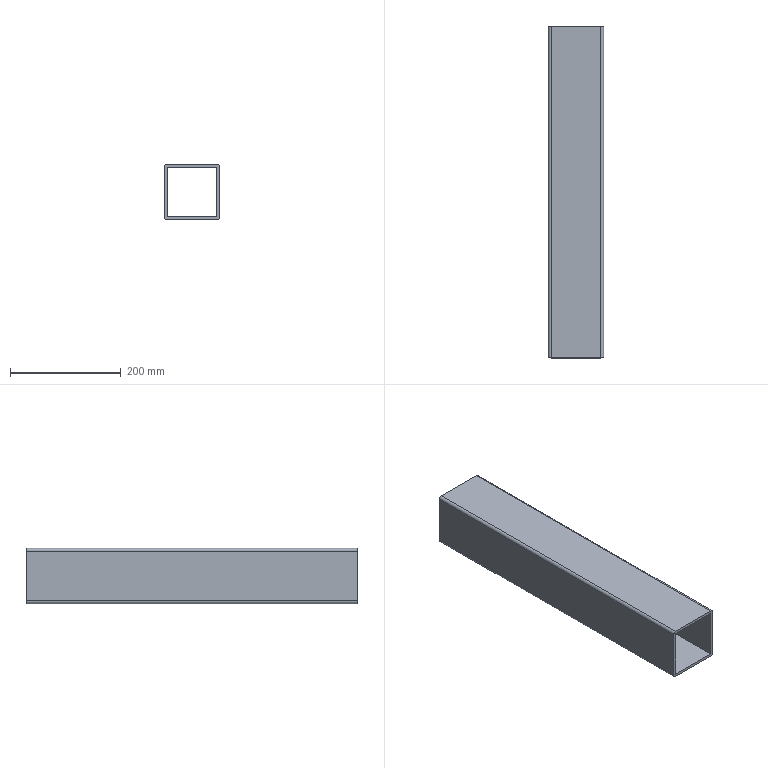Component | NX | TUBO_INFERIOR | 1 solid | 14 faces | box 100 x 600 x 100 mm | volume 1127124 mm3 | plane 10 | cylinder 4 | commonest cylinder face diameters 10 x4
STEP:
#1=CARTESIAN_POINT('',(0.,0.,0.));
#2=DIRECTION('',(0.,0.,1.));
#3=DIRECTION('',(1.,0.,0.));
#4=AXIS2_PLACEMENT_3D('',#1,#2,#3);
#5=CARTESIAN_POINT('',(0.,-34.8,155.));
#6=VERTEX_POINT('',#5);
#7=CARTESIAN_POINT('',(0.,-34.8,65.));
#8=VERTEX_POINT('',#7);
#9=CARTESIAN_POINT('',(0.,-34.8,160.));
#10=DIRECTION('',(0.,0.,-1.));
#11=VECTOR('',#10,1.);
#12=LINE('',#9,#11);
#13=CARTESIAN_POINT('',(0.,-634.8,160.));
#14=DIRECTION('',(1.,0.,0.));
#15=DIRECTION('',(0.,0.,-1.));
#16=AXIS2_PLACEMENT_3D('',#13,#14,#15);
#17=PLANE('',#16);
#18=CARTESIAN_POINT('',(0.,600.));
#19=DIRECTION('',(1.,0.));
#20=VECTOR('',#19,1.);
#21=LINE('',#18,#20);
#22=(GEOMETRIC_REPRESENTATION_CONTEXT(2)PARAMETRIC_REPRESENTATION_CONTEXT()REPRESENTATION_CONTEXT('',''));
#23=DEFINITIONAL_REPRESENTATION('',(#21),#22);
#24=PCURVE('',#17,#23);
#25=CARTESIAN_POINT('',(0.,-34.8,60.));
#26=DIRECTION('',(0.,-1.,0.));
#27=DIRECTION('',(0.,0.,-1.));
#28=AXIS2_PLACEMENT_3D('',#25,#26,#27);
#29=PLANE('',#28);
#30=CARTESIAN_POINT('',(-100.,-0.));
#31=DIRECTION('',(1.,0.));
#32=VECTOR('',#31,1.);
#33=LINE('',#30,#32);
#34=(GEOMETRIC_REPRESENTATION_CONTEXT(2)PARAMETRIC_REPRESENTATION_CONTEXT()REPRESENTATION_CONTEXT('',''));
#35=DEFINITIONAL_REPRESENTATION('',(#33),#34);
#36=PCURVE('',#29,#35);
#37=SURFACE_CURVE('',#12,(#24,#36),.PCURVE_S1.);
#38=EDGE_CURVE('',#6,#8,#37,.T.);
#39=ORIENTED_EDGE('',*,*,#38,.T.);
#40=CARTESIAN_POINT('',(0.,-634.8,65.));
#41=VERTEX_POINT('',#40);
#42=CARTESIAN_POINT('',(0.,-634.8,65.));
#43=DIRECTION('',(0.,-1.,0.));
#44=VECTOR('',#43,1.);
#45=LINE('',#42,#44);
#46=CARTESIAN_POINT('',(95.,0.));
#47=DIRECTION('',(0.,-1.));
#48=VECTOR('',#47,1.);
#49=LINE('',#46,#48);
#50=(GEOMETRIC_REPRESENTATION_CONTEXT(2)PARAMETRIC_REPRESENTATION_CONTEXT()REPRESENTATION_CONTEXT('',''));
#51=DEFINITIONAL_REPRESENTATION('',(#49),#50);
#52=PCURVE('',#17,#51);
#53=CARTESIAN_POINT('',(5.,-634.8,65.));
#54=DIRECTION('',(0.,1.,0.));
#55=DIRECTION('',(0.,0.,1.));
#56=AXIS2_PLACEMENT_3D('',#53,#54,#55);
#57=CYLINDRICAL_SURFACE('',#56,5.);
#58=CARTESIAN_POINT('',(4.712,0.));
#59=DIRECTION('',(0.,-1.));
#60=VECTOR('',#59,1.);
#61=LINE('',#58,#60);
#62=(GEOMETRIC_REPRESENTATION_CONTEXT(2)PARAMETRIC_REPRESENTATION_CONTEXT()REPRESENTATION_CONTEXT('',''));
#63=DEFINITIONAL_REPRESENTATION('',(#61),#62);
#64=PCURVE('',#57,#63);
#65=SURFACE_CURVE('',#45,(#52,#64),.PCURVE_S1.);
#66=EDGE_CURVE('',#8,#41,#65,.T.);
#67=ORIENTED_EDGE('',*,*,#66,.T.);
#68=CARTESIAN_POINT('',(0.,-634.8,155.));
#69=VERTEX_POINT('',#68);
#70=CARTESIAN_POINT('',(0.,-634.8,160.));
#71=DIRECTION('',(0.,0.,-1.));
#72=VECTOR('',#71,1.);
#73=LINE('',#70,#72);
#74=CARTESIAN_POINT('',(0.,0.));
#75=DIRECTION('',(1.,0.));
#76=VECTOR('',#75,1.);
#77=LINE('',#74,#76);
#78=(GEOMETRIC_REPRESENTATION_CONTEXT(2)PARAMETRIC_REPRESENTATION_CONTEXT()REPRESENTATION_CONTEXT('',''));
#79=DEFINITIONAL_REPRESENTATION('',(#77),#78);
#80=PCURVE('',#17,#79);
#81=CARTESIAN_POINT('',(0.,-634.8,60.));
#82=DIRECTION('',(0.,-1.,0.));
#83=DIRECTION('',(0.,0.,-1.));
#84=AXIS2_PLACEMENT_3D('',#81,#82,#83);
#85=PLANE('',#84);
#86=CARTESIAN_POINT('',(-100.,-0.));
#87=DIRECTION('',(1.,0.));
#88=VECTOR('',#87,1.);
#89=LINE('',#86,#88);
#90=(GEOMETRIC_REPRESENTATION_CONTEXT(2)PARAMETRIC_REPRESENTATION_CONTEXT()REPRESENTATION_CONTEXT('',''));
#91=DEFINITIONAL_REPRESENTATION('',(#89),#90);
#92=PCURVE('',#85,#91);
#93=SURFACE_CURVE('',#73,(#80,#92),.PCURVE_S1.);
#94=EDGE_CURVE('',#69,#41,#93,.T.);
#95=ORIENTED_EDGE('',*,*,#94,.F.);
#96=CARTESIAN_POINT('',(0.,-634.8,155.));
#97=DIRECTION('',(0.,1.,0.));
#98=VECTOR('',#97,1.);
#99=LINE('',#96,#98);
#100=CARTESIAN_POINT('',(5.,0.));
#101=DIRECTION('',(0.,1.));
#102=VECTOR('',#101,1.);
#103=LINE('',#100,#102);
#104=(GEOMETRIC_REPRESENTATION_CONTEXT(2)PARAMETRIC_REPRESENTATION_CONTEXT()REPRESENTATION_CONTEXT('',''));
#105=DEFINITIONAL_REPRESENTATION('',(#103),#104);
#106=PCURVE('',#17,#105);
#107=CARTESIAN_POINT('',(5.,-634.8,155.));
#108=DIRECTION('',(0.,1.,0.));
#109=DIRECTION('',(0.,0.,1.));
#110=AXIS2_PLACEMENT_3D('',#107,#108,#109);
#111=CYLINDRICAL_SURFACE('',#110,5.);
#112=CARTESIAN_POINT('',(4.712,0.));
#113=DIRECTION('',(0.,1.));
#114=VECTOR('',#113,1.);
#115=LINE('',#112,#114);
#116=(GEOMETRIC_REPRESENTATION_CONTEXT(2)PARAMETRIC_REPRESENTATION_CONTEXT()REPRESENTATION_CONTEXT('',''));
#117=DEFINITIONAL_REPRESENTATION('',(#115),#116);
#118=PCURVE('',#111,#117);
#119=SURFACE_CURVE('',#99,(#106,#118),.PCURVE_S1.);
#120=EDGE_CURVE('',#69,#6,#119,.T.);
#121=ORIENTED_EDGE('',*,*,#120,.T.);
#122=EDGE_LOOP('',(#39,#67,#95,#121));
#123=FACE_BOUND('',#122,.T.);
#124=ADVANCED_FACE('',(#123),#17,.F.);
#125=CARTESIAN_POINT('',(5.,-634.8,60.));
#126=VERTEX_POINT('',#125);
#127=CARTESIAN_POINT('',(95.,-634.8,60.));
#128=VERTEX_POINT('',#127);
#129=CARTESIAN_POINT('',(0.,-634.8,60.));
#130=DIRECTION('',(1.,0.,0.));
#131=VECTOR('',#130,1.);
#132=LINE('',#129,#131);
#133=CARTESIAN_POINT('',(0.,-634.8,60.));
#134=DIRECTION('',(-0.,0.,1.));
#135=DIRECTION('',(1.,0.,0.));
#136=AXIS2_PLACEMENT_3D('',#133,#134,#135);
#137=PLANE('',#136);
#138=CARTESIAN_POINT('',(0.,0.));
#139=DIRECTION('',(1.,0.));
#140=VECTOR('',#139,1.);
#141=LINE('',#138,#140);
#142=(GEOMETRIC_REPRESENTATION_CONTEXT(2)PARAMETRIC_REPRESENTATION_CONTEXT()REPRESENTATION_CONTEXT('',''));
#143=DEFINITIONAL_REPRESENTATION('',(#141),#142);
#144=PCURVE('',#137,#143);
#145=CARTESIAN_POINT('',(0.,0.));
#146=DIRECTION('',(-0.,1.));
#147=VECTOR('',#146,1.);
#148=LINE('',#145,#147);
#149=(GEOMETRIC_REPRESENTATION_CONTEXT(2)PARAMETRIC_REPRESENTATION_CONTEXT()REPRESENTATION_CONTEXT('',''));
#150=DEFINITIONAL_REPRESENTATION('',(#148),#149);
#151=PCURVE('',#85,#150);
#152=SURFACE_CURVE('',#132,(#144,#151),.PCURVE_S1.);
#153=EDGE_CURVE('',#126,#128,#152,.T.);
#154=ORIENTED_EDGE('',*,*,#153,.F.);
#155=CARTESIAN_POINT('',(5.,-34.8,60.));
#156=VERTEX_POINT('',#155);
#157=CARTESIAN_POINT('',(5.,-634.8,60.));
#158=DIRECTION('',(0.,1.,0.));
#159=VECTOR('',#158,1.);
#160=LINE('',#157,#159);
#161=CARTESIAN_POINT('',(5.,0.));
#162=DIRECTION('',(0.,1.));
#163=VECTOR('',#162,1.);
#164=LINE('',#161,#163);
#165=(GEOMETRIC_REPRESENTATION_CONTEXT(2)PARAMETRIC_REPRESENTATION_CONTEXT()REPRESENTATION_CONTEXT('',''));
#166=DEFINITIONAL_REPRESENTATION('',(#164),#165);
#167=PCURVE('',#137,#166);
#168=CARTESIAN_POINT('',(3.142,0.));
#169=DIRECTION('',(0.,1.));
#170=VECTOR('',#169,1.);
#171=LINE('',#168,#170);
#172=(GEOMETRIC_REPRESENTATION_CONTEXT(2)PARAMETRIC_REPRESENTATION_CONTEXT()REPRESENTATION_CONTEXT('',''));
#173=DEFINITIONAL_REPRESENTATION('',(#171),#172);
#174=PCURVE('',#57,#173);
#175=SURFACE_CURVE('',#160,(#167,#174),.PCURVE_S1.);
#176=EDGE_CURVE('',#126,#156,#175,.T.);
#177=ORIENTED_EDGE('',*,*,#176,.T.);
#178=CARTESIAN_POINT('',(95.,-34.8,60.));
#179=VERTEX_POINT('',#178);
#180=CARTESIAN_POINT('',(0.,-34.8,60.));
#181=DIRECTION('',(1.,0.,0.));
#182=VECTOR('',#181,1.);
#183=LINE('',#180,#182);
#184=CARTESIAN_POINT('',(0.,600.));
#185=DIRECTION('',(1.,0.));
#186=VECTOR('',#185,1.);
#187=LINE('',#184,#186);
#188=(GEOMETRIC_REPRESENTATION_CONTEXT(2)PARAMETRIC_REPRESENTATION_CONTEXT()REPRESENTATION_CONTEXT('',''));
#189=DEFINITIONAL_REPRESENTATION('',(#187),#188);
#190=PCURVE('',#137,#189);
#191=CARTESIAN_POINT('',(0.,0.));
#192=DIRECTION('',(-0.,1.));
#193=VECTOR('',#192,1.);
#194=LINE('',#191,#193);
#195=(GEOMETRIC_REPRESENTATION_CONTEXT(2)PARAMETRIC_REPRESENTATION_CONTEXT()REPRESENTATION_CONTEXT('',''));
#196=DEFINITIONAL_REPRESENTATION('',(#194),#195);
#197=PCURVE('',#29,#196);
#198=SURFACE_CURVE('',#183,(#190,#197),.PCURVE_S1.);
#199=EDGE_CURVE('',#156,#179,#198,.T.);
#200=ORIENTED_EDGE('',*,*,#199,.T.);
#201=CARTESIAN_POINT('',(95.,-634.8,60.));
#202=DIRECTION('',(0.,-1.,0.));
#203=VECTOR('',#202,1.);
#204=LINE('',#201,#203);
#205=CARTESIAN_POINT('',(95.,0.));
#206=DIRECTION('',(0.,-1.));
#207=VECTOR('',#206,1.);
#208=LINE('',#205,#207);
#209=(GEOMETRIC_REPRESENTATION_CONTEXT(2)PARAMETRIC_REPRESENTATION_CONTEXT()REPRESENTATION_CONTEXT('',''));
#210=DEFINITIONAL_REPRESENTATION('',(#208),#209);
#211=PCURVE('',#137,#210);
#212=CARTESIAN_POINT('',(95.,-634.8,65.));
#213=DIRECTION('',(0.,1.,0.));
#214=DIRECTION('',(0.,0.,1.));
#215=AXIS2_PLACEMENT_3D('',#212,#213,#214);
#216=CYLINDRICAL_SURFACE('',#215,5.);
#217=CARTESIAN_POINT('',(3.142,0.));
#218=DIRECTION('',(0.,-1.));
#219=VECTOR('',#218,1.);
#220=LINE('',#217,#219);
#221=(GEOMETRIC_REPRESENTATION_CONTEXT(2)PARAMETRIC_REPRESENTATION_CONTEXT()REPRESENTATION_CONTEXT('',''));
#222=DEFINITIONAL_REPRESENTATION('',(#220),#221);
#223=PCURVE('',#216,#222);
#224=SURFACE_CURVE('',#204,(#211,#223),.PCURVE_S1.);
#225=EDGE_CURVE('',#179,#128,#224,.T.);
#226=ORIENTED_EDGE('',*,*,#225,.T.);
#227=EDGE_LOOP('',(#154,#177,#200,#226));
#228=FACE_BOUND('',#227,.T.);
#229=ADVANCED_FACE('',(#228),#137,.F.);
#230=CARTESIAN_POINT('',(100.,-634.8,65.));
#231=VERTEX_POINT('',#230);
#232=CARTESIAN_POINT('',(100.,-634.8,155.));
#233=VERTEX_POINT('',#232);
#234=CARTESIAN_POINT('',(100.,-634.8,60.));
#235=DIRECTION('',(-0.,0.,1.));
#236=VECTOR('',#235,1.);
#237=LINE('',#234,#236);
#238=CARTESIAN_POINT('',(100.,-634.8,60.));
#239=DIRECTION('',(-1.,0.,-0.));
#240=DIRECTION('',(-0.,0.,1.));
#241=AXIS2_PLACEMENT_3D('',#238,#239,#240);
#242=PLANE('',#241);
#243=CARTESIAN_POINT('',(0.,0.));
#244=DIRECTION('',(1.,0.));
#245=VECTOR('',#244,1.);
#246=LINE('',#243,#245);
#247=(GEOMETRIC_REPRESENTATION_CONTEXT(2)PARAMETRIC_REPRESENTATION_CONTEXT()REPRESENTATION_CONTEXT('',''));
#248=DEFINITIONAL_REPRESENTATION('',(#246),#247);
#249=PCURVE('',#242,#248);
#250=CARTESIAN_POINT('',(0.,100.));
#251=DIRECTION('',(-1.,-0.));
#252=VECTOR('',#251,1.);
#253=LINE('',#250,#252);
#254=(GEOMETRIC_REPRESENTATION_CONTEXT(2)PARAMETRIC_REPRESENTATION_CONTEXT()REPRESENTATION_CONTEXT('',''));
#255=DEFINITIONAL_REPRESENTATION('',(#253),#254);
#256=PCURVE('',#85,#255);
#257=SURFACE_CURVE('',#237,(#249,#256),.PCURVE_S1.);
#258=EDGE_CURVE('',#231,#233,#257,.T.);
#259=ORIENTED_EDGE('',*,*,#258,.F.);
#260=CARTESIAN_POINT('',(100.,-34.8,65.));
#261=VERTEX_POINT('',#260);
#262=CARTESIAN_POINT('',(100.,-634.8,65.));
#263=DIRECTION('',(0.,1.,0.));
#264=VECTOR('',#263,1.);
#265=LINE('',#262,#264);
#266=CARTESIAN_POINT('',(5.,0.));
#267=DIRECTION('',(0.,1.));
#268=VECTOR('',#267,1.);
#269=LINE('',#266,#268);
#270=(GEOMETRIC_REPRESENTATION_CONTEXT(2)PARAMETRIC_REPRESENTATION_CONTEXT()REPRESENTATION_CONTEXT('',''));
#271=DEFINITIONAL_REPRESENTATION('',(#269),#270);
#272=PCURVE('',#242,#271);
#273=CARTESIAN_POINT('',(1.571,0.));
#274=DIRECTION('',(0.,1.));
#275=VECTOR('',#274,1.);
#276=LINE('',#273,#275);
#277=(GEOMETRIC_REPRESENTATION_CONTEXT(2)PARAMETRIC_REPRESENTATION_CONTEXT()REPRESENTATION_CONTEXT('',''));
#278=DEFINITIONAL_REPRESENTATION('',(#276),#277);
#279=PCURVE('',#216,#278);
#280=SURFACE_CURVE('',#265,(#272,#279),.PCURVE_S1.);
#281=EDGE_CURVE('',#231,#261,#280,.T.);
#282=ORIENTED_EDGE('',*,*,#281,.T.);
#283=CARTESIAN_POINT('',(100.,-34.8,155.));
#284=VERTEX_POINT('',#283);
#285=CARTESIAN_POINT('',(100.,-34.8,60.));
#286=DIRECTION('',(-0.,0.,1.));
#287=VECTOR('',#286,1.);
#288=LINE('',#285,#287);
#289=CARTESIAN_POINT('',(0.,600.));
#290=DIRECTION('',(1.,0.));
#291=VECTOR('',#290,1.);
#292=LINE('',#289,#291);
#293=(GEOMETRIC_REPRESENTATION_CONTEXT(2)PARAMETRIC_REPRESENTATION_CONTEXT()REPRESENTATION_CONTEXT('',''));
#294=DEFINITIONAL_REPRESENTATION('',(#292),#293);
#295=PCURVE('',#242,#294);
#296=CARTESIAN_POINT('',(0.,100.));
#297=DIRECTION('',(-1.,-0.));
#298=VECTOR('',#297,1.);
#299=LINE('',#296,#298);
#300=(GEOMETRIC_REPRESENTATION_CONTEXT(2)PARAMETRIC_REPRESENTATION_CONTEXT()REPRESENTATION_CONTEXT('',''));
#301=DEFINITIONAL_REPRESENTATION('',(#299),#300);
#302=PCURVE('',#29,#301);
#303=SURFACE_CURVE('',#288,(#295,#302),.PCURVE_S1.);
#304=EDGE_CURVE('',#261,#284,#303,.T.);
#305=ORIENTED_EDGE('',*,*,#304,.T.);
#306=CARTESIAN_POINT('',(100.,-634.8,155.));
#307=DIRECTION('',(0.,-1.,0.));
#308=VECTOR('',#307,1.);
#309=LINE('',#306,#308);
#310=CARTESIAN_POINT('',(95.,0.));
#311=DIRECTION('',(0.,-1.));
#312=VECTOR('',#311,1.);
#313=LINE('',#310,#312);
#314=(GEOMETRIC_REPRESENTATION_CONTEXT(2)PARAMETRIC_REPRESENTATION_CONTEXT()REPRESENTATION_CONTEXT('',''));
#315=DEFINITIONAL_REPRESENTATION('',(#313),#314);
#316=PCURVE('',#242,#315);
#317=CARTESIAN_POINT('',(95.,-634.8,155.));
#318=DIRECTION('',(0.,1.,0.));
#319=DIRECTION('',(0.,0.,1.));
#320=AXIS2_PLACEMENT_3D('',#317,#318,#319);
#321=CYLINDRICAL_SURFACE('',#320,5.);
#322=CARTESIAN_POINT('',(1.571,0.));
#323=DIRECTION('',(0.,-1.));
#324=VECTOR('',#323,1.);
#325=LINE('',#322,#324);
#326=(GEOMETRIC_REPRESENTATION_CONTEXT(2)PARAMETRIC_REPRESENTATION_CONTEXT()REPRESENTATION_CONTEXT('',''));
#327=DEFINITIONAL_REPRESENTATION('',(#325),#326);
#328=PCURVE('',#321,#327);
#329=SURFACE_CURVE('',#309,(#316,#328),.PCURVE_S1.);
#330=EDGE_CURVE('',#284,#233,#329,.T.);
#331=ORIENTED_EDGE('',*,*,#330,.T.);
#332=EDGE_LOOP('',(#259,#282,#305,#331));
#333=FACE_BOUND('',#332,.T.);
#334=ADVANCED_FACE('',(#333),#242,.F.);
#335=CARTESIAN_POINT('',(95.,-34.8,160.));
#336=VERTEX_POINT('',#335);
#337=CARTESIAN_POINT('',(5.,-34.8,160.));
#338=VERTEX_POINT('',#337);
#339=CARTESIAN_POINT('',(100.,-34.8,160.));
#340=DIRECTION('',(-1.,0.,-0.));
#341=VECTOR('',#340,1.);
#342=LINE('',#339,#341);
#343=CARTESIAN_POINT('',(100.,-634.8,160.));
#344=DIRECTION('',(0.,0.,-1.));
#345=DIRECTION('',(-1.,0.,-0.));
#346=AXIS2_PLACEMENT_3D('',#343,#344,#345);
#347=PLANE('',#346);
#348=CARTESIAN_POINT('',(0.,600.));
#349=DIRECTION('',(1.,0.));
#350=VECTOR('',#349,1.);
#351=LINE('',#348,#350);
#352=(GEOMETRIC_REPRESENTATION_CONTEXT(2)PARAMETRIC_REPRESENTATION_CONTEXT()REPRESENTATION_CONTEXT('',''));
#353=DEFINITIONAL_REPRESENTATION('',(#351),#352);
#354=PCURVE('',#347,#353);
#355=CARTESIAN_POINT('',(-100.,100.));
#356=DIRECTION('',(0.,-1.));
#357=VECTOR('',#356,1.);
#358=LINE('',#355,#357);
#359=(GEOMETRIC_REPRESENTATION_CONTEXT(2)PARAMETRIC_REPRESENTATION_CONTEXT()REPRESENTATION_CONTEXT('',''));
#360=DEFINITIONAL_REPRESENTATION('',(#358),#359);
#361=PCURVE('',#29,#360);
#362=SURFACE_CURVE('',#342,(#354,#361),.PCURVE_S1.);
#363=EDGE_CURVE('',#336,#338,#362,.T.);
#364=ORIENTED_EDGE('',*,*,#363,.T.);
#365=CARTESIAN_POINT('',(5.,-634.8,160.));
#366=VERTEX_POINT('',#365);
#367=CARTESIAN_POINT('',(5.,-634.8,160.));
#368=DIRECTION('',(0.,-1.,0.));
#369=VECTOR('',#368,1.);
#370=LINE('',#367,#369);
#371=CARTESIAN_POINT('',(95.,0.));
#372=DIRECTION('',(0.,-1.));
#373=VECTOR('',#372,1.);
#374=LINE('',#371,#373);
#375=(GEOMETRIC_REPRESENTATION_CONTEXT(2)PARAMETRIC_REPRESENTATION_CONTEXT()REPRESENTATION_CONTEXT('',''));
#376=DEFINITIONAL_REPRESENTATION('',(#374),#375);
#377=PCURVE('',#347,#376);
#378=CARTESIAN_POINT('',(6.283,0.));
#379=DIRECTION('',(0.,-1.));
#380=VECTOR('',#379,1.);
#381=LINE('',#378,#380);
#382=(GEOMETRIC_REPRESENTATION_CONTEXT(2)PARAMETRIC_REPRESENTATION_CONTEXT()REPRESENTATION_CONTEXT('',''));
#383=DEFINITIONAL_REPRESENTATION('',(#381),#382);
#384=PCURVE('',#111,#383);
#385=SURFACE_CURVE('',#370,(#377,#384),.PCURVE_S1.);
#386=EDGE_CURVE('',#338,#366,#385,.T.);
#387=ORIENTED_EDGE('',*,*,#386,.T.);
#388=CARTESIAN_POINT('',(95.,-634.8,160.));
#389=VERTEX_POINT('',#388);
#390=CARTESIAN_POINT('',(100.,-634.8,160.));
#391=DIRECTION('',(-1.,0.,-0.));
#392=VECTOR('',#391,1.);
#393=LINE('',#390,#392);
#394=CARTESIAN_POINT('',(0.,0.));
#395=DIRECTION('',(1.,0.));
#396=VECTOR('',#395,1.);
#397=LINE('',#394,#396);
#398=(GEOMETRIC_REPRESENTATION_CONTEXT(2)PARAMETRIC_REPRESENTATION_CONTEXT()REPRESENTATION_CONTEXT('',''));
#399=DEFINITIONAL_REPRESENTATION('',(#397),#398);
#400=PCURVE('',#347,#399);
#401=CARTESIAN_POINT('',(-100.,100.));
#402=DIRECTION('',(0.,-1.));
#403=VECTOR('',#402,1.);
#404=LINE('',#401,#403);
#405=(GEOMETRIC_REPRESENTATION_CONTEXT(2)PARAMETRIC_REPRESENTATION_CONTEXT()REPRESENTATION_CONTEXT('',''));
#406=DEFINITIONAL_REPRESENTATION('',(#404),#405);
#407=PCURVE('',#85,#406);
#408=SURFACE_CURVE('',#393,(#400,#407),.PCURVE_S1.);
#409=EDGE_CURVE('',#389,#366,#408,.T.);
#410=ORIENTED_EDGE('',*,*,#409,.F.);
#411=CARTESIAN_POINT('',(95.,-634.8,160.));
#412=DIRECTION('',(0.,1.,0.));
#413=VECTOR('',#412,1.);
#414=LINE('',#411,#413);
#415=CARTESIAN_POINT('',(5.,0.));
#416=DIRECTION('',(0.,1.));
#417=VECTOR('',#416,1.);
#418=LINE('',#415,#417);
#419=(GEOMETRIC_REPRESENTATION_CONTEXT(2)PARAMETRIC_REPRESENTATION_CONTEXT()REPRESENTATION_CONTEXT('',''));
#420=DEFINITIONAL_REPRESENTATION('',(#418),#419);
#421=PCURVE('',#347,#420);
#422=CARTESIAN_POINT('',(0.,0.));
#423=DIRECTION('',(0.,1.));
#424=VECTOR('',#423,1.);
#425=LINE('',#422,#424);
#426=(GEOMETRIC_REPRESENTATION_CONTEXT(2)PARAMETRIC_REPRESENTATION_CONTEXT()REPRESENTATION_CONTEXT('',''));
#427=DEFINITIONAL_REPRESENTATION('',(#425),#426);
#428=PCURVE('',#321,#427);
#429=SURFACE_CURVE('',#414,(#421,#428),.PCURVE_S1.);
#430=EDGE_CURVE('',#389,#336,#429,.T.);
#431=ORIENTED_EDGE('',*,*,#430,.T.);
#432=EDGE_LOOP('',(#364,#387,#410,#431));
#433=FACE_BOUND('',#432,.T.);
#434=ADVANCED_FACE('',(#433),#347,.F.);
#435=CARTESIAN_POINT('',(5.,-634.8,155.));
#436=VERTEX_POINT('',#435);
#437=CARTESIAN_POINT('',(5.,-634.8,65.));
#438=VERTEX_POINT('',#437);
#439=CARTESIAN_POINT('',(5.,-634.8,160.));
#440=DIRECTION('',(0.,0.,-1.));
#441=VECTOR('',#440,1.);
#442=LINE('',#439,#441);
#443=CARTESIAN_POINT('',(-100.,5.));
#444=DIRECTION('',(1.,0.));
#445=VECTOR('',#444,1.);
#446=LINE('',#443,#445);
#447=(GEOMETRIC_REPRESENTATION_CONTEXT(2)PARAMETRIC_REPRESENTATION_CONTEXT()REPRESENTATION_CONTEXT('',''));
#448=DEFINITIONAL_REPRESENTATION('',(#446),#447);
#449=PCURVE('',#85,#448);
#450=CARTESIAN_POINT('',(5.,-634.8,160.));
#451=DIRECTION('',(1.,0.,0.));
#452=DIRECTION('',(0.,0.,-1.));
#453=AXIS2_PLACEMENT_3D('',#450,#451,#452);
#454=PLANE('',#453);
#455=CARTESIAN_POINT('',(0.,0.));
#456=DIRECTION('',(1.,0.));
#457=VECTOR('',#456,1.);
#458=LINE('',#455,#457);
#459=(GEOMETRIC_REPRESENTATION_CONTEXT(2)PARAMETRIC_REPRESENTATION_CONTEXT()REPRESENTATION_CONTEXT('',''));
#460=DEFINITIONAL_REPRESENTATION('',(#458),#459);
#461=PCURVE('',#454,#460);
#462=SURFACE_CURVE('',#442,(#449,#461),.PCURVE_S1.);
#463=EDGE_CURVE('',#436,#438,#462,.T.);
#464=ORIENTED_EDGE('',*,*,#463,.F.);
#465=CARTESIAN_POINT('',(95.,-634.8,155.));
#466=VERTEX_POINT('',#465);
#467=CARTESIAN_POINT('',(100.,-634.8,155.));
#468=DIRECTION('',(-1.,0.,-0.));
#469=VECTOR('',#468,1.);
#470=LINE('',#467,#469);
#471=CARTESIAN_POINT('',(-95.,100.));
#472=DIRECTION('',(0.,-1.));
#473=VECTOR('',#472,1.);
#474=LINE('',#471,#473);
#475=(GEOMETRIC_REPRESENTATION_CONTEXT(2)PARAMETRIC_REPRESENTATION_CONTEXT()REPRESENTATION_CONTEXT('',''));
#476=DEFINITIONAL_REPRESENTATION('',(#474),#475);
#477=PCURVE('',#85,#476);
#478=CARTESIAN_POINT('',(100.,-634.8,155.));
#479=DIRECTION('',(0.,0.,-1.));
#480=DIRECTION('',(-1.,0.,-0.));
#481=AXIS2_PLACEMENT_3D('',#478,#479,#480);
#482=PLANE('',#481);
#483=CARTESIAN_POINT('',(0.,0.));
#484=DIRECTION('',(1.,0.));
#485=VECTOR('',#484,1.);
#486=LINE('',#483,#485);
#487=(GEOMETRIC_REPRESENTATION_CONTEXT(2)PARAMETRIC_REPRESENTATION_CONTEXT()REPRESENTATION_CONTEXT('',''));
#488=DEFINITIONAL_REPRESENTATION('',(#486),#487);
#489=PCURVE('',#482,#488);
#490=SURFACE_CURVE('',#470,(#477,#489),.PCURVE_S1.);
#491=EDGE_CURVE('',#466,#436,#490,.T.);
#492=ORIENTED_EDGE('',*,*,#491,.F.);
#493=CARTESIAN_POINT('',(95.,-634.8,65.));
#494=VERTEX_POINT('',#493);
#495=CARTESIAN_POINT('',(95.,-634.8,60.));
#496=DIRECTION('',(-0.,0.,1.));
#497=VECTOR('',#496,1.);
#498=LINE('',#495,#497);
#499=CARTESIAN_POINT('',(0.,95.));
#500=DIRECTION('',(-1.,-0.));
#501=VECTOR('',#500,1.);
#502=LINE('',#499,#501);
#503=(GEOMETRIC_REPRESENTATION_CONTEXT(2)PARAMETRIC_REPRESENTATION_CONTEXT()REPRESENTATION_CONTEXT('',''));
#504=DEFINITIONAL_REPRESENTATION('',(#502),#503);
#505=PCURVE('',#85,#504);
#506=CARTESIAN_POINT('',(95.,-634.8,60.));
#507=DIRECTION('',(-1.,0.,-0.));
#508=DIRECTION('',(-0.,0.,1.));
#509=AXIS2_PLACEMENT_3D('',#506,#507,#508);
#510=PLANE('',#509);
#511=CARTESIAN_POINT('',(0.,0.));
#512=DIRECTION('',(1.,0.));
#513=VECTOR('',#512,1.);
#514=LINE('',#511,#513);
#515=(GEOMETRIC_REPRESENTATION_CONTEXT(2)PARAMETRIC_REPRESENTATION_CONTEXT()REPRESENTATION_CONTEXT('',''));
#516=DEFINITIONAL_REPRESENTATION('',(#514),#515);
#517=PCURVE('',#510,#516);
#518=SURFACE_CURVE('',#498,(#505,#517),.PCURVE_S1.);
#519=EDGE_CURVE('',#494,#466,#518,.T.);
#520=ORIENTED_EDGE('',*,*,#519,.F.);
#521=CARTESIAN_POINT('',(0.,-634.8,65.));
#522=DIRECTION('',(1.,0.,0.));
#523=VECTOR('',#522,1.);
#524=LINE('',#521,#523);
#525=CARTESIAN_POINT('',(-5.,-0.));
#526=DIRECTION('',(-0.,1.));
#527=VECTOR('',#526,1.);
#528=LINE('',#525,#527);
#529=(GEOMETRIC_REPRESENTATION_CONTEXT(2)PARAMETRIC_REPRESENTATION_CONTEXT()REPRESENTATION_CONTEXT('',''));
#530=DEFINITIONAL_REPRESENTATION('',(#528),#529);
#531=PCURVE('',#85,#530);
#532=CARTESIAN_POINT('',(0.,-634.8,65.));
#533=DIRECTION('',(-0.,0.,1.));
#534=DIRECTION('',(1.,0.,0.));
#535=AXIS2_PLACEMENT_3D('',#532,#533,#534);
#536=PLANE('',#535);
#537=CARTESIAN_POINT('',(0.,0.));
#538=DIRECTION('',(1.,0.));
#539=VECTOR('',#538,1.);
#540=LINE('',#537,#539);
#541=(GEOMETRIC_REPRESENTATION_CONTEXT(2)PARAMETRIC_REPRESENTATION_CONTEXT()REPRESENTATION_CONTEXT('',''));
#542=DEFINITIONAL_REPRESENTATION('',(#540),#541);
#543=PCURVE('',#536,#542);
#544=SURFACE_CURVE('',#524,(#531,#543),.PCURVE_S1.);
#545=EDGE_CURVE('',#438,#494,#544,.T.);
#546=ORIENTED_EDGE('',*,*,#545,.F.);
#547=EDGE_LOOP('',(#464,#492,#520,#546));
#548=FACE_BOUND('',#547,.T.);
#549=ORIENTED_EDGE('',*,*,#94,.T.);
#550=CARTESIAN_POINT('',(5.,-634.8,65.));
#551=DIRECTION('',(0.,-1.,0.));
#552=DIRECTION('',(0.,0.,-1.));
#553=AXIS2_PLACEMENT_3D('',#550,#551,#552);
#554=CIRCLE('',#553,5.);
#555=CARTESIAN_POINT('',(-5.,5.));
#556=DIRECTION('',(1.,0.));
#557=AXIS2_PLACEMENT_2D('',#555,#556);
#558=CIRCLE('',#557,5.);
#559=(GEOMETRIC_REPRESENTATION_CONTEXT(2)PARAMETRIC_REPRESENTATION_CONTEXT()REPRESENTATION_CONTEXT('',''));
#560=DEFINITIONAL_REPRESENTATION('',(#558),#559);
#561=PCURVE('',#85,#560);
#562=CARTESIAN_POINT('',(9.425,0.));
#563=DIRECTION('',(-1.,0.));
#564=VECTOR('',#563,1.);
#565=LINE('',#562,#564);
#566=(GEOMETRIC_REPRESENTATION_CONTEXT(2)PARAMETRIC_REPRESENTATION_CONTEXT()REPRESENTATION_CONTEXT('',''));
#567=DEFINITIONAL_REPRESENTATION('',(#565),#566);
#568=PCURVE('',#57,#567);
#569=SURFACE_CURVE('',#554,(#561,#568),.PCURVE_S1.);
#570=EDGE_CURVE('',#41,#126,#569,.T.);
#571=ORIENTED_EDGE('',*,*,#570,.T.);
#572=ORIENTED_EDGE('',*,*,#153,.T.);
#573=CARTESIAN_POINT('',(95.,-634.8,65.));
#574=DIRECTION('',(0.,-1.,0.));
#575=DIRECTION('',(0.,0.,-1.));
#576=AXIS2_PLACEMENT_3D('',#573,#574,#575);
#577=CIRCLE('',#576,5.);
#578=CARTESIAN_POINT('',(-5.,95.));
#579=DIRECTION('',(1.,0.));
#580=AXIS2_PLACEMENT_2D('',#578,#579);
#581=CIRCLE('',#580,5.);
#582=(GEOMETRIC_REPRESENTATION_CONTEXT(2)PARAMETRIC_REPRESENTATION_CONTEXT()REPRESENTATION_CONTEXT('',''));
#583=DEFINITIONAL_REPRESENTATION('',(#581),#582);
#584=PCURVE('',#85,#583);
#585=CARTESIAN_POINT('',(3.142,0.));
#586=DIRECTION('',(-1.,0.));
#587=VECTOR('',#586,1.);
#588=LINE('',#585,#587);
#589=(GEOMETRIC_REPRESENTATION_CONTEXT(2)PARAMETRIC_REPRESENTATION_CONTEXT()REPRESENTATION_CONTEXT('',''));
#590=DEFINITIONAL_REPRESENTATION('',(#588),#589);
#591=PCURVE('',#216,#590);
#592=SURFACE_CURVE('',#577,(#584,#591),.PCURVE_S1.);
#593=EDGE_CURVE('',#128,#231,#592,.T.);
#594=ORIENTED_EDGE('',*,*,#593,.T.);
#595=ORIENTED_EDGE('',*,*,#258,.T.);
#596=CARTESIAN_POINT('',(95.,-634.8,155.));
#597=DIRECTION('',(0.,-1.,0.));
#598=DIRECTION('',(0.,0.,-1.));
#599=AXIS2_PLACEMENT_3D('',#596,#597,#598);
#600=CIRCLE('',#599,5.);
#601=CARTESIAN_POINT('',(-95.,95.));
#602=DIRECTION('',(1.,0.));
#603=AXIS2_PLACEMENT_2D('',#601,#602);
#604=CIRCLE('',#603,5.);
#605=(GEOMETRIC_REPRESENTATION_CONTEXT(2)PARAMETRIC_REPRESENTATION_CONTEXT()REPRESENTATION_CONTEXT('',''));
#606=DEFINITIONAL_REPRESENTATION('',(#604),#605);
#607=PCURVE('',#85,#606);
#608=CARTESIAN_POINT('',(3.142,0.));
#609=DIRECTION('',(-1.,0.));
#610=VECTOR('',#609,1.);
#611=LINE('',#608,#610);
#612=(GEOMETRIC_REPRESENTATION_CONTEXT(2)PARAMETRIC_REPRESENTATION_CONTEXT()REPRESENTATION_CONTEXT('',''));
#613=DEFINITIONAL_REPRESENTATION('',(#611),#612);
#614=PCURVE('',#321,#613);
#615=SURFACE_CURVE('',#600,(#607,#614),.PCURVE_S1.);
#616=EDGE_CURVE('',#233,#389,#615,.T.);
#617=ORIENTED_EDGE('',*,*,#616,.T.);
#618=ORIENTED_EDGE('',*,*,#409,.T.);
#619=CARTESIAN_POINT('',(5.,-634.8,155.));
#620=DIRECTION('',(0.,-1.,0.));
#621=DIRECTION('',(0.,0.,-1.));
#622=AXIS2_PLACEMENT_3D('',#619,#620,#621);
#623=CIRCLE('',#622,5.);
#624=CARTESIAN_POINT('',(-95.,5.));
#625=DIRECTION('',(1.,0.));
#626=AXIS2_PLACEMENT_2D('',#624,#625);
#627=CIRCLE('',#626,5.);
#628=(GEOMETRIC_REPRESENTATION_CONTEXT(2)PARAMETRIC_REPRESENTATION_CONTEXT()REPRESENTATION_CONTEXT('',''));
#629=DEFINITIONAL_REPRESENTATION('',(#627),#628);
#630=PCURVE('',#85,#629);
#631=CARTESIAN_POINT('',(9.425,0.));
#632=DIRECTION('',(-1.,0.));
#633=VECTOR('',#632,1.);
#634=LINE('',#631,#633);
#635=(GEOMETRIC_REPRESENTATION_CONTEXT(2)PARAMETRIC_REPRESENTATION_CONTEXT()REPRESENTATION_CONTEXT('',''));
#636=DEFINITIONAL_REPRESENTATION('',(#634),#635);
#637=PCURVE('',#111,#636);
#638=SURFACE_CURVE('',#623,(#630,#637),.PCURVE_S1.);
#639=EDGE_CURVE('',#366,#69,#638,.T.);
#640=ORIENTED_EDGE('',*,*,#639,.T.);
#641=EDGE_LOOP('',(#549,#571,#572,#594,#595,#617,#618,#640));
#642=FACE_BOUND('',#641,.T.);
#643=ADVANCED_FACE('',(#548,#642),#85,.T.);
#644=CARTESIAN_POINT('',(5.,-34.8,155.));
#645=VERTEX_POINT('',#644);
#646=CARTESIAN_POINT('',(5.,-34.8,65.));
#647=VERTEX_POINT('',#646);
#648=CARTESIAN_POINT('',(5.,-34.8,160.));
#649=DIRECTION('',(0.,0.,-1.));
#650=VECTOR('',#649,1.);
#651=LINE('',#648,#650);
#652=CARTESIAN_POINT('',(-100.,5.));
#653=DIRECTION('',(1.,0.));
#654=VECTOR('',#653,1.);
#655=LINE('',#652,#654);
#656=(GEOMETRIC_REPRESENTATION_CONTEXT(2)PARAMETRIC_REPRESENTATION_CONTEXT()REPRESENTATION_CONTEXT('',''));
#657=DEFINITIONAL_REPRESENTATION('',(#655),#656);
#658=PCURVE('',#29,#657);
#659=CARTESIAN_POINT('',(0.,600.));
#660=DIRECTION('',(1.,0.));
#661=VECTOR('',#660,1.);
#662=LINE('',#659,#661);
#663=(GEOMETRIC_REPRESENTATION_CONTEXT(2)PARAMETRIC_REPRESENTATION_CONTEXT()REPRESENTATION_CONTEXT('',''));
#664=DEFINITIONAL_REPRESENTATION('',(#662),#663);
#665=PCURVE('',#454,#664);
#666=SURFACE_CURVE('',#651,(#658,#665),.PCURVE_S1.);
#667=EDGE_CURVE('',#645,#647,#666,.T.);
#668=ORIENTED_EDGE('',*,*,#667,.T.);
#669=CARTESIAN_POINT('',(95.,-34.8,65.));
#670=VERTEX_POINT('',#669);
#671=CARTESIAN_POINT('',(0.,-34.8,65.));
#672=DIRECTION('',(1.,0.,0.));
#673=VECTOR('',#672,1.);
#674=LINE('',#671,#673);
#675=CARTESIAN_POINT('',(-5.,-0.));
#676=DIRECTION('',(-0.,1.));
#677=VECTOR('',#676,1.);
#678=LINE('',#675,#677);
#679=(GEOMETRIC_REPRESENTATION_CONTEXT(2)PARAMETRIC_REPRESENTATION_CONTEXT()REPRESENTATION_CONTEXT('',''));
#680=DEFINITIONAL_REPRESENTATION('',(#678),#679);
#681=PCURVE('',#29,#680);
#682=CARTESIAN_POINT('',(0.,600.));
#683=DIRECTION('',(1.,0.));
#684=VECTOR('',#683,1.);
#685=LINE('',#682,#684);
#686=(GEOMETRIC_REPRESENTATION_CONTEXT(2)PARAMETRIC_REPRESENTATION_CONTEXT()REPRESENTATION_CONTEXT('',''));
#687=DEFINITIONAL_REPRESENTATION('',(#685),#686);
#688=PCURVE('',#536,#687);
#689=SURFACE_CURVE('',#674,(#681,#688),.PCURVE_S1.);
#690=EDGE_CURVE('',#647,#670,#689,.T.);
#691=ORIENTED_EDGE('',*,*,#690,.T.);
#692=CARTESIAN_POINT('',(95.,-34.8,155.));
#693=VERTEX_POINT('',#692);
#694=CARTESIAN_POINT('',(95.,-34.8,60.));
#695=DIRECTION('',(-0.,0.,1.));
#696=VECTOR('',#695,1.);
#697=LINE('',#694,#696);
#698=CARTESIAN_POINT('',(0.,95.));
#699=DIRECTION('',(-1.,-0.));
#700=VECTOR('',#699,1.);
#701=LINE('',#698,#700);
#702=(GEOMETRIC_REPRESENTATION_CONTEXT(2)PARAMETRIC_REPRESENTATION_CONTEXT()REPRESENTATION_CONTEXT('',''));
#703=DEFINITIONAL_REPRESENTATION('',(#701),#702);
#704=PCURVE('',#29,#703);
#705=CARTESIAN_POINT('',(0.,600.));
#706=DIRECTION('',(1.,0.));
#707=VECTOR('',#706,1.);
#708=LINE('',#705,#707);
#709=(GEOMETRIC_REPRESENTATION_CONTEXT(2)PARAMETRIC_REPRESENTATION_CONTEXT()REPRESENTATION_CONTEXT('',''));
#710=DEFINITIONAL_REPRESENTATION('',(#708),#709);
#711=PCURVE('',#510,#710);
#712=SURFACE_CURVE('',#697,(#704,#711),.PCURVE_S1.);
#713=EDGE_CURVE('',#670,#693,#712,.T.);
#714=ORIENTED_EDGE('',*,*,#713,.T.);
#715=CARTESIAN_POINT('',(100.,-34.8,155.));
#716=DIRECTION('',(-1.,0.,-0.));
#717=VECTOR('',#716,1.);
#718=LINE('',#715,#717);
#719=CARTESIAN_POINT('',(-95.,100.));
#720=DIRECTION('',(0.,-1.));
#721=VECTOR('',#720,1.);
#722=LINE('',#719,#721);
#723=(GEOMETRIC_REPRESENTATION_CONTEXT(2)PARAMETRIC_REPRESENTATION_CONTEXT()REPRESENTATION_CONTEXT('',''));
#724=DEFINITIONAL_REPRESENTATION('',(#722),#723);
#725=PCURVE('',#29,#724);
#726=CARTESIAN_POINT('',(0.,600.));
#727=DIRECTION('',(1.,0.));
#728=VECTOR('',#727,1.);
#729=LINE('',#726,#728);
#730=(GEOMETRIC_REPRESENTATION_CONTEXT(2)PARAMETRIC_REPRESENTATION_CONTEXT()REPRESENTATION_CONTEXT('',''));
#731=DEFINITIONAL_REPRESENTATION('',(#729),#730);
#732=PCURVE('',#482,#731);
#733=SURFACE_CURVE('',#718,(#725,#732),.PCURVE_S1.);
#734=EDGE_CURVE('',#693,#645,#733,.T.);
#735=ORIENTED_EDGE('',*,*,#734,.T.);
#736=EDGE_LOOP('',(#668,#691,#714,#735));
#737=FACE_BOUND('',#736,.T.);
#738=ORIENTED_EDGE('',*,*,#199,.F.);
#739=CARTESIAN_POINT('',(5.,-34.8,65.));
#740=DIRECTION('',(0.,1.,0.));
#741=DIRECTION('',(0.,0.,-1.));
#742=AXIS2_PLACEMENT_3D('',#739,#740,#741);
#743=CIRCLE('',#742,5.);
#744=CARTESIAN_POINT('',(0.,5.));
#745=CARTESIAN_POINT('',(0.,-3.66));
#746=CARTESIAN_POINT('',(-7.5,0.6699));
#747=CARTESIAN_POINT('',(-15.,5.));
#748=CARTESIAN_POINT('',(-7.5,9.33));
#749=CARTESIAN_POINT('',(-0.,13.66));
#750=CARTESIAN_POINT('',(0.,5.));
#751=(BOUNDED_CURVE()B_SPLINE_CURVE(2,(#744,#745,#746,#747,#748,#749,#750),.UNSPECIFIED.,.T.,.F.)B_SPLINE_CURVE_WITH_KNOTS((1,2,2,2,2,1),(-2.094,0.,2.094,4.189,6.283,8.378),.UNSPECIFIED.)CURVE()GEOMETRIC_REPRESENTATION_ITEM()RATIONAL_B_SPLINE_CURVE((1.,0.5,1.,0.5,1.,0.5,1.))REPRESENTATION_ITEM(''));
#752=(GEOMETRIC_REPRESENTATION_CONTEXT(2)PARAMETRIC_REPRESENTATION_CONTEXT()REPRESENTATION_CONTEXT('',''));
#753=DEFINITIONAL_REPRESENTATION('',(#751),#752);
#754=PCURVE('',#29,#753);
#755=CARTESIAN_POINT('',(3.142,600.));
#756=DIRECTION('',(1.,0.));
#757=VECTOR('',#756,1.);
#758=LINE('',#755,#757);
#759=(GEOMETRIC_REPRESENTATION_CONTEXT(2)PARAMETRIC_REPRESENTATION_CONTEXT()REPRESENTATION_CONTEXT('',''));
#760=DEFINITIONAL_REPRESENTATION('',(#758),#759);
#761=PCURVE('',#57,#760);
#762=SURFACE_CURVE('',#743,(#754,#761),.PCURVE_S1.);
#763=EDGE_CURVE('',#156,#8,#762,.T.);
#764=ORIENTED_EDGE('',*,*,#763,.T.);
#765=ORIENTED_EDGE('',*,*,#38,.F.);
#766=CARTESIAN_POINT('',(5.,-34.8,155.));
#767=DIRECTION('',(0.,1.,0.));
#768=DIRECTION('',(0.,0.,-1.));
#769=AXIS2_PLACEMENT_3D('',#766,#767,#768);
#770=CIRCLE('',#769,5.);
#771=CARTESIAN_POINT('',(-90.,5.));
#772=CARTESIAN_POINT('',(-90.,-3.66));
#773=CARTESIAN_POINT('',(-97.5,0.6699));
#774=CARTESIAN_POINT('',(-105.,5.));
#775=CARTESIAN_POINT('',(-97.5,9.33));
#776=CARTESIAN_POINT('',(-90.,13.66));
#777=CARTESIAN_POINT('',(-90.,5.));
#778=(BOUNDED_CURVE()B_SPLINE_CURVE(2,(#771,#772,#773,#774,#775,#776,#777),.UNSPECIFIED.,.T.,.F.)B_SPLINE_CURVE_WITH_KNOTS((1,2,2,2,2,1),(-2.094,0.,2.094,4.189,6.283,8.378),.UNSPECIFIED.)CURVE()GEOMETRIC_REPRESENTATION_ITEM()RATIONAL_B_SPLINE_CURVE((1.,0.5,1.,0.5,1.,0.5,1.))REPRESENTATION_ITEM(''));
#779=(GEOMETRIC_REPRESENTATION_CONTEXT(2)PARAMETRIC_REPRESENTATION_CONTEXT()REPRESENTATION_CONTEXT('',''));
#780=DEFINITIONAL_REPRESENTATION('',(#778),#779);
#781=PCURVE('',#29,#780);
#782=CARTESIAN_POINT('',(3.142,600.));
#783=DIRECTION('',(1.,0.));
#784=VECTOR('',#783,1.);
#785=LINE('',#782,#784);
#786=(GEOMETRIC_REPRESENTATION_CONTEXT(2)PARAMETRIC_REPRESENTATION_CONTEXT()REPRESENTATION_CONTEXT('',''));
#787=DEFINITIONAL_REPRESENTATION('',(#785),#786);
#788=PCURVE('',#111,#787);
#789=SURFACE_CURVE('',#770,(#781,#788),.PCURVE_S1.);
#790=EDGE_CURVE('',#6,#338,#789,.T.);
#791=ORIENTED_EDGE('',*,*,#790,.T.);
#792=ORIENTED_EDGE('',*,*,#363,.F.);
#793=CARTESIAN_POINT('',(95.,-34.8,155.));
#794=DIRECTION('',(0.,1.,0.));
#795=DIRECTION('',(0.,0.,-1.));
#796=AXIS2_PLACEMENT_3D('',#793,#794,#795);
#797=CIRCLE('',#796,5.);
#798=CARTESIAN_POINT('',(-90.,95.));
#799=CARTESIAN_POINT('',(-90.,86.34));
#800=CARTESIAN_POINT('',(-97.5,90.67));
#801=CARTESIAN_POINT('',(-105.,95.));
#802=CARTESIAN_POINT('',(-97.5,99.33));
#803=CARTESIAN_POINT('',(-90.,103.66));
#804=CARTESIAN_POINT('',(-90.,95.));
#805=(BOUNDED_CURVE()B_SPLINE_CURVE(2,(#798,#799,#800,#801,#802,#803,#804),.UNSPECIFIED.,.T.,.F.)B_SPLINE_CURVE_WITH_KNOTS((1,2,2,2,2,1),(-2.094,0.,2.094,4.189,6.283,8.378),.UNSPECIFIED.)CURVE()GEOMETRIC_REPRESENTATION_ITEM()RATIONAL_B_SPLINE_CURVE((1.,0.5,1.,0.5,1.,0.5,1.))REPRESENTATION_ITEM(''));
#806=(GEOMETRIC_REPRESENTATION_CONTEXT(2)PARAMETRIC_REPRESENTATION_CONTEXT()REPRESENTATION_CONTEXT('',''));
#807=DEFINITIONAL_REPRESENTATION('',(#805),#806);
#808=PCURVE('',#29,#807);
#809=CARTESIAN_POINT('',(-3.142,600.));
#810=DIRECTION('',(1.,0.));
#811=VECTOR('',#810,1.);
#812=LINE('',#809,#811);
#813=(GEOMETRIC_REPRESENTATION_CONTEXT(2)PARAMETRIC_REPRESENTATION_CONTEXT()REPRESENTATION_CONTEXT('',''));
#814=DEFINITIONAL_REPRESENTATION('',(#812),#813);
#815=PCURVE('',#321,#814);
#816=SURFACE_CURVE('',#797,(#808,#815),.PCURVE_S1.);
#817=EDGE_CURVE('',#336,#284,#816,.T.);
#818=ORIENTED_EDGE('',*,*,#817,.T.);
#819=ORIENTED_EDGE('',*,*,#304,.F.);
#820=CARTESIAN_POINT('',(95.,-34.8,65.));
#821=DIRECTION('',(0.,1.,0.));
#822=DIRECTION('',(0.,0.,-1.));
#823=AXIS2_PLACEMENT_3D('',#820,#821,#822);
#824=CIRCLE('',#823,5.);
#825=CARTESIAN_POINT('',(0.,95.));
#826=CARTESIAN_POINT('',(0.,86.34));
#827=CARTESIAN_POINT('',(-7.5,90.67));
#828=CARTESIAN_POINT('',(-15.,95.));
#829=CARTESIAN_POINT('',(-7.5,99.33));
#830=CARTESIAN_POINT('',(-0.,103.66));
#831=CARTESIAN_POINT('',(0.,95.));
#832=(BOUNDED_CURVE()B_SPLINE_CURVE(2,(#825,#826,#827,#828,#829,#830,#831),.UNSPECIFIED.,.T.,.F.)B_SPLINE_CURVE_WITH_KNOTS((1,2,2,2,2,1),(-2.094,0.,2.094,4.189,6.283,8.378),.UNSPECIFIED.)CURVE()GEOMETRIC_REPRESENTATION_ITEM()RATIONAL_B_SPLINE_CURVE((1.,0.5,1.,0.5,1.,0.5,1.))REPRESENTATION_ITEM(''));
#833=(GEOMETRIC_REPRESENTATION_CONTEXT(2)PARAMETRIC_REPRESENTATION_CONTEXT()REPRESENTATION_CONTEXT('',''));
#834=DEFINITIONAL_REPRESENTATION('',(#832),#833);
#835=PCURVE('',#29,#834);
#836=CARTESIAN_POINT('',(-3.142,600.));
#837=DIRECTION('',(1.,0.));
#838=VECTOR('',#837,1.);
#839=LINE('',#836,#838);
#840=(GEOMETRIC_REPRESENTATION_CONTEXT(2)PARAMETRIC_REPRESENTATION_CONTEXT()REPRESENTATION_CONTEXT('',''));
#841=DEFINITIONAL_REPRESENTATION('',(#839),#840);
#842=PCURVE('',#216,#841);
#843=SURFACE_CURVE('',#824,(#835,#842),.PCURVE_S1.);
#844=EDGE_CURVE('',#261,#179,#843,.T.);
#845=ORIENTED_EDGE('',*,*,#844,.T.);
#846=EDGE_LOOP('',(#738,#764,#765,#791,#792,#818,#819,#845));
#847=FACE_BOUND('',#846,.T.);
#848=ADVANCED_FACE('',(#737,#847),#29,.F.);
#849=ORIENTED_EDGE('',*,*,#570,.F.);
#850=ORIENTED_EDGE('',*,*,#66,.F.);
#851=ORIENTED_EDGE('',*,*,#763,.F.);
#852=ORIENTED_EDGE('',*,*,#176,.F.);
#853=EDGE_LOOP('',(#849,#850,#851,#852));
#854=FACE_BOUND('',#853,.T.);
#855=ADVANCED_FACE('',(#854),#57,.T.);
#856=ORIENTED_EDGE('',*,*,#593,.F.);
#857=ORIENTED_EDGE('',*,*,#225,.F.);
#858=ORIENTED_EDGE('',*,*,#844,.F.);
#859=ORIENTED_EDGE('',*,*,#281,.F.);
#860=EDGE_LOOP('',(#856,#857,#858,#859));
#861=FACE_BOUND('',#860,.T.);
#862=ADVANCED_FACE('',(#861),#216,.T.);
#863=ORIENTED_EDGE('',*,*,#639,.F.);
#864=ORIENTED_EDGE('',*,*,#386,.F.);
#865=ORIENTED_EDGE('',*,*,#790,.F.);
#866=ORIENTED_EDGE('',*,*,#120,.F.);
#867=EDGE_LOOP('',(#863,#864,#865,#866));
#868=FACE_BOUND('',#867,.T.);
#869=ADVANCED_FACE('',(#868),#111,.T.);
#870=ORIENTED_EDGE('',*,*,#616,.F.);
#871=ORIENTED_EDGE('',*,*,#330,.F.);
#872=ORIENTED_EDGE('',*,*,#817,.F.);
#873=ORIENTED_EDGE('',*,*,#430,.F.);
#874=EDGE_LOOP('',(#870,#871,#872,#873));
#875=FACE_BOUND('',#874,.T.);
#876=ADVANCED_FACE('',(#875),#321,.T.);
#877=ORIENTED_EDGE('',*,*,#667,.F.);
#878=CARTESIAN_POINT('',(5.,-634.8,155.));
#879=DIRECTION('',(0.,-1.,0.));
#880=VECTOR('',#879,1.);
#881=LINE('',#878,#880);
#882=CARTESIAN_POINT('',(5.,0.));
#883=DIRECTION('',(0.,-1.));
#884=VECTOR('',#883,1.);
#885=LINE('',#882,#884);
#886=(GEOMETRIC_REPRESENTATION_CONTEXT(2)PARAMETRIC_REPRESENTATION_CONTEXT()REPRESENTATION_CONTEXT('',''));
#887=DEFINITIONAL_REPRESENTATION('',(#885),#886);
#888=PCURVE('',#454,#887);
#889=CARTESIAN_POINT('',(95.,0.));
#890=DIRECTION('',(0.,-1.));
#891=VECTOR('',#890,1.);
#892=LINE('',#889,#891);
#893=(GEOMETRIC_REPRESENTATION_CONTEXT(2)PARAMETRIC_REPRESENTATION_CONTEXT()REPRESENTATION_CONTEXT('',''));
#894=DEFINITIONAL_REPRESENTATION('',(#892),#893);
#895=PCURVE('',#482,#894);
#896=SURFACE_CURVE('',#881,(#888,#895),.PCURVE_S1.);
#897=EDGE_CURVE('',#645,#436,#896,.T.);
#898=ORIENTED_EDGE('',*,*,#897,.T.);
#899=ORIENTED_EDGE('',*,*,#463,.T.);
#900=CARTESIAN_POINT('',(5.,-634.8,65.));
#901=DIRECTION('',(0.,-1.,0.));
#902=VECTOR('',#901,1.);
#903=LINE('',#900,#902);
#904=CARTESIAN_POINT('',(95.,0.));
#905=DIRECTION('',(0.,-1.));
#906=VECTOR('',#905,1.);
#907=LINE('',#904,#906);
#908=(GEOMETRIC_REPRESENTATION_CONTEXT(2)PARAMETRIC_REPRESENTATION_CONTEXT()REPRESENTATION_CONTEXT('',''));
#909=DEFINITIONAL_REPRESENTATION('',(#907),#908);
#910=PCURVE('',#454,#909);
#911=CARTESIAN_POINT('',(5.,0.));
#912=DIRECTION('',(0.,-1.));
#913=VECTOR('',#912,1.);
#914=LINE('',#911,#913);
#915=(GEOMETRIC_REPRESENTATION_CONTEXT(2)PARAMETRIC_REPRESENTATION_CONTEXT()REPRESENTATION_CONTEXT('',''));
#916=DEFINITIONAL_REPRESENTATION('',(#914),#915);
#917=PCURVE('',#536,#916);
#918=SURFACE_CURVE('',#903,(#910,#917),.PCURVE_S1.);
#919=EDGE_CURVE('',#647,#438,#918,.T.);
#920=ORIENTED_EDGE('',*,*,#919,.F.);
#921=EDGE_LOOP('',(#877,#898,#899,#920));
#922=FACE_BOUND('',#921,.T.);
#923=ADVANCED_FACE('',(#922),#454,.T.);
#924=ORIENTED_EDGE('',*,*,#545,.T.);
#925=CARTESIAN_POINT('',(95.,-634.8,65.));
#926=DIRECTION('',(0.,-1.,0.));
#927=VECTOR('',#926,1.);
#928=LINE('',#925,#927);
#929=CARTESIAN_POINT('',(95.,0.));
#930=DIRECTION('',(0.,-1.));
#931=VECTOR('',#930,1.);
#932=LINE('',#929,#931);
#933=(GEOMETRIC_REPRESENTATION_CONTEXT(2)PARAMETRIC_REPRESENTATION_CONTEXT()REPRESENTATION_CONTEXT('',''));
#934=DEFINITIONAL_REPRESENTATION('',(#932),#933);
#935=PCURVE('',#536,#934);
#936=CARTESIAN_POINT('',(5.,0.));
#937=DIRECTION('',(0.,-1.));
#938=VECTOR('',#937,1.);
#939=LINE('',#936,#938);
#940=(GEOMETRIC_REPRESENTATION_CONTEXT(2)PARAMETRIC_REPRESENTATION_CONTEXT()REPRESENTATION_CONTEXT('',''));
#941=DEFINITIONAL_REPRESENTATION('',(#939),#940);
#942=PCURVE('',#510,#941);
#943=SURFACE_CURVE('',#928,(#935,#942),.PCURVE_S1.);
#944=EDGE_CURVE('',#670,#494,#943,.T.);
#945=ORIENTED_EDGE('',*,*,#944,.F.);
#946=ORIENTED_EDGE('',*,*,#690,.F.);
#947=ORIENTED_EDGE('',*,*,#919,.T.);
#948=EDGE_LOOP('',(#924,#945,#946,#947));
#949=FACE_BOUND('',#948,.T.);
#950=ADVANCED_FACE('',(#949),#536,.T.);
#951=ORIENTED_EDGE('',*,*,#519,.T.);
#952=CARTESIAN_POINT('',(95.,-634.8,155.));
#953=DIRECTION('',(0.,-1.,0.));
#954=VECTOR('',#953,1.);
#955=LINE('',#952,#954);
#956=CARTESIAN_POINT('',(95.,0.));
#957=DIRECTION('',(0.,-1.));
#958=VECTOR('',#957,1.);
#959=LINE('',#956,#958);
#960=(GEOMETRIC_REPRESENTATION_CONTEXT(2)PARAMETRIC_REPRESENTATION_CONTEXT()REPRESENTATION_CONTEXT('',''));
#961=DEFINITIONAL_REPRESENTATION('',(#959),#960);
#962=PCURVE('',#510,#961);
#963=CARTESIAN_POINT('',(5.,0.));
#964=DIRECTION('',(0.,-1.));
#965=VECTOR('',#964,1.);
#966=LINE('',#963,#965);
#967=(GEOMETRIC_REPRESENTATION_CONTEXT(2)PARAMETRIC_REPRESENTATION_CONTEXT()REPRESENTATION_CONTEXT('',''));
#968=DEFINITIONAL_REPRESENTATION('',(#966),#967);
#969=PCURVE('',#482,#968);
#970=SURFACE_CURVE('',#955,(#962,#969),.PCURVE_S1.);
#971=EDGE_CURVE('',#693,#466,#970,.T.);
#972=ORIENTED_EDGE('',*,*,#971,.F.);
#973=ORIENTED_EDGE('',*,*,#713,.F.);
#974=ORIENTED_EDGE('',*,*,#944,.T.);
#975=EDGE_LOOP('',(#951,#972,#973,#974));
#976=FACE_BOUND('',#975,.T.);
#977=ADVANCED_FACE('',(#976),#510,.T.);
#978=ORIENTED_EDGE('',*,*,#734,.F.);
#979=ORIENTED_EDGE('',*,*,#971,.T.);
#980=ORIENTED_EDGE('',*,*,#491,.T.);
#981=ORIENTED_EDGE('',*,*,#897,.F.);
#982=EDGE_LOOP('',(#978,#979,#980,#981));
#983=FACE_BOUND('',#982,.T.);
#984=ADVANCED_FACE('',(#983),#482,.T.);
#985=CLOSED_SHELL('',(#124,#229,#334,#434,#643,#848,#855,#862,#869,#876,#923,#950,#977,#984));
#986=MANIFOLD_SOLID_BREP('',#985);
#987=(LENGTH_UNIT()NAMED_UNIT(*)SI_UNIT(.MILLI.,.METRE.));
#988=UNCERTAINTY_MEASURE_WITH_UNIT(LENGTH_MEASURE(0.0000001),#987,'','');
#989=(NAMED_UNIT(*)PLANE_ANGLE_UNIT()SI_UNIT($,.RADIAN.));
#990=(NAMED_UNIT(*)SI_UNIT($,.STERADIAN.)SOLID_ANGLE_UNIT());
#991=(GEOMETRIC_REPRESENTATION_CONTEXT(3)GLOBAL_UNCERTAINTY_ASSIGNED_CONTEXT((#988))GLOBAL_UNIT_ASSIGNED_CONTEXT((#987,#989,#990))REPRESENTATION_CONTEXT('',''));
#992=ADVANCED_BREP_SHAPE_REPRESENTATION('',(#4,#986),#991);